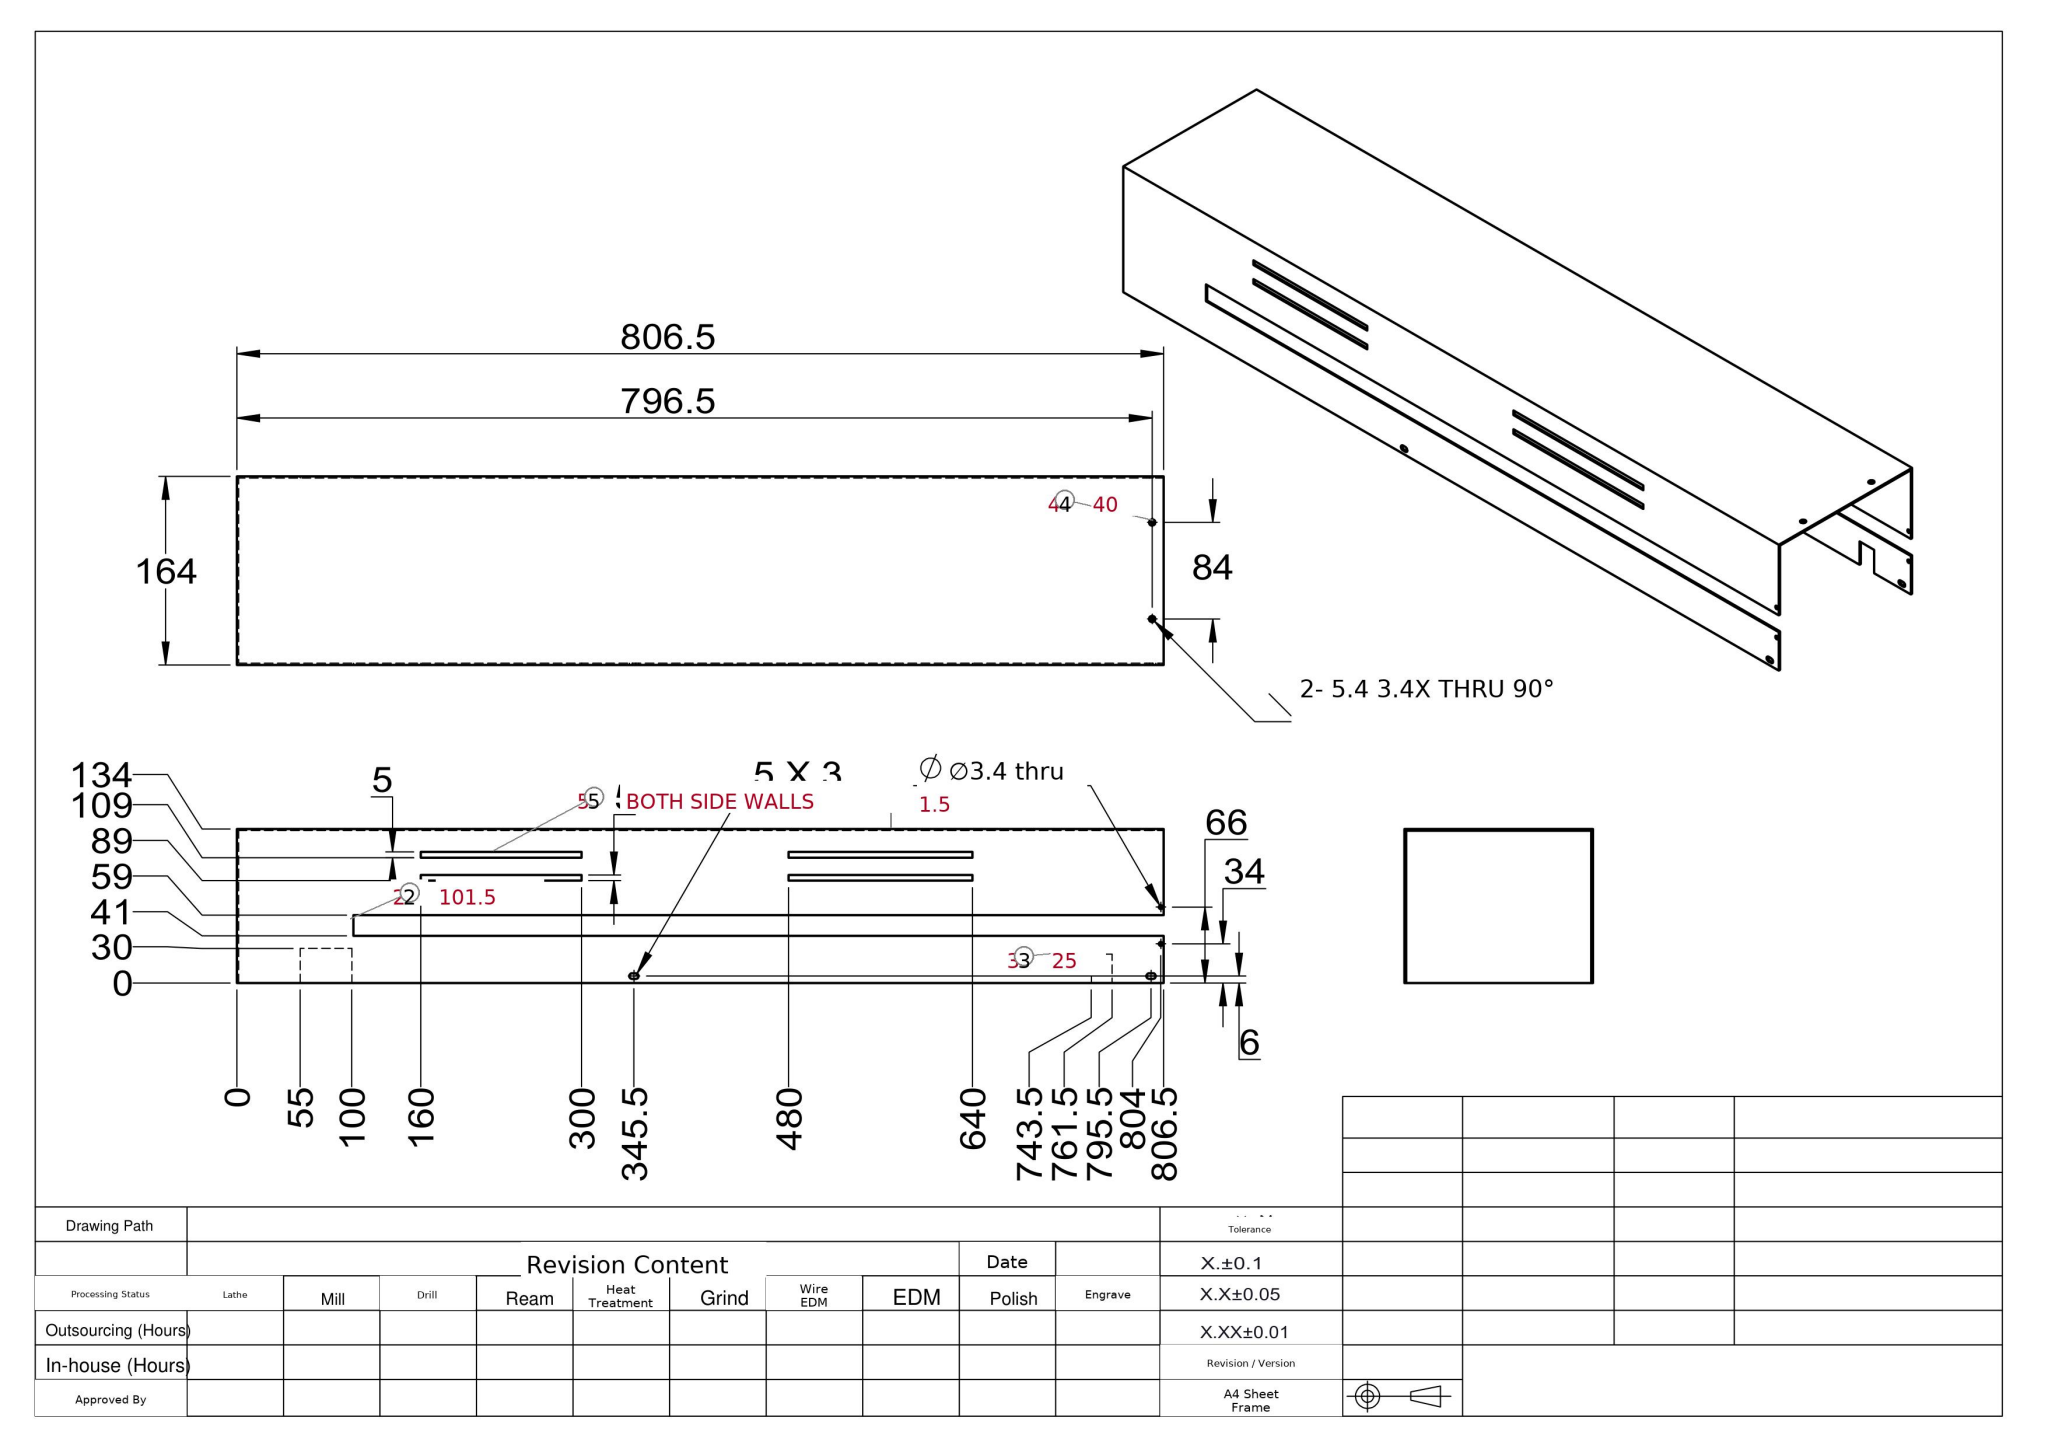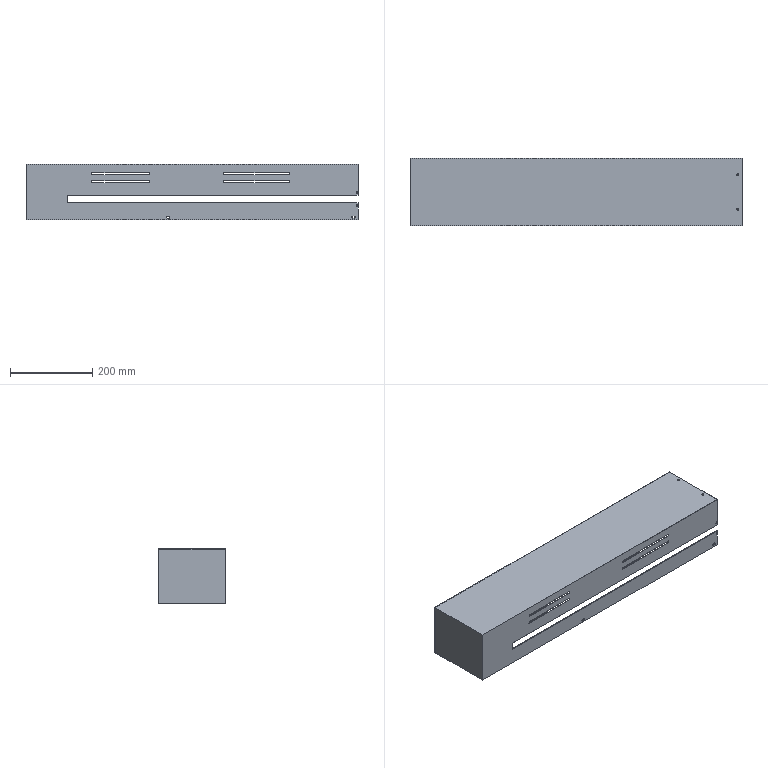Part | SolidWorks | mm | 1 solid | 90 faces | box 806.5 x 164 x 134 mm | volume 500909 mm3 | plane 66 | cylinder 20 | cone 4 | commonest cylinder face diameters 3.4 x12 5 x8
build123d program:
from build123d import *

# Parameters (mm, degrees)
SKETCH1_W           = 806.5
SKETCH1_H           = 164
BOSS_EXTRUDE1_DEPTH = 134
SKETCH2_W           = 805
SKETCH2_H           = 161
CUT_EXTRUDE1_DEPTH  = 834.843
SKETCH3_W           = 806.5
SKETCH3_H           = 164
BOSS_EXTRUDE2_DEPTH = 1.5
SKETCH4_W           = 705
SKETCH4_H           = 18
CUT_EXTRUDE2_DEPTH  = 834.843
SKETCH5_W           = 800
SKETCH5_H           = 5
CUT_EXTRUDE3_DEPTH  = 834.843
LPATTERN1_COUNT     = 2
LPATTERN1_PITCH     = 20
CUT_EXTRUDE4_DEPTH  = 834.843
LPATTERN2_COUNT     = 3
LPATTERN2_PITCH     = 450
SKETCH8_R           = 1.7
CUT_EXTRUDE5_DEPTH  = 1.5
CHAMFER1_SIZE       = 1
SKETCH9_W           = 45
SKETCH9_H           = 30
CUT_EXTRUDE6_DEPTH  = 10
SKETCH10_W          = 18
SKETCH10_H          = 25
CUT_EXTRUDE7_DEPTH  = 10
SKETCH11_W          = 180
SKETCH11_H          = 25
SKETCH11_W_2        = 166.5
BOSS_EXTRUDE4_DEPTH = 1.5
SKETCH12_W          = 180
SKETCH12_H          = 25
SKETCH12_W_2        = 166.5
BOSS_EXTRUDE5_DEPTH = 1.5
SKETCH14_R          = 1.7
CUT_EXTRUDE8_DEPTH  = 834.843


with BuildPart() as part:
    # Sketch1 → Boss-Extrude1 (new body)
    with BuildSketch(Plane.XY):
        with Locations((403.25, 82)):
            Rectangle(SKETCH1_W, SKETCH1_H)
    extrude(amount=BOSS_EXTRUDE1_DEPTH)

    # Sketch2 → Cut-Extrude1 (cut, through all)
    with BuildSketch(Plane.XY.offset(134)):
        with Locations((404, 82)):
            Rectangle(SKETCH2_W, SKETCH2_H)
    extrude(amount=-CUT_EXTRUDE1_DEPTH, mode=Mode.SUBTRACT)

    # Sketch3 → Boss-Extrude2 (add)
    with BuildSketch(Plane.XY.offset(134)):
        with Locations((403.25, 82)):
            Rectangle(SKETCH3_W, SKETCH3_H)
    extrude(amount=-BOSS_EXTRUDE2_DEPTH)

    # Sketch4 → Cut-Extrude2 (cut, through all)
    with BuildSketch(Plane(origin=(0, 164, 0), x_dir=(1, 0, 0), z_dir=(0, 1, 0))):
        with Locations((454, -50)):
            Rectangle(SKETCH4_W, SKETCH4_H)
    extrude(amount=-CUT_EXTRUDE2_DEPTH, mode=Mode.SUBTRACT)

    # Sketch5 → Cut-Extrude3 (cut, through all)
    with BuildSketch(Plane.XZ):
        with Locations((560, 111.5)):
            Rectangle(SKETCH5_W, SKETCH5_H)
    cut_extrude3 = extrude(amount=-CUT_EXTRUDE3_DEPTH, mode=Mode.SUBTRACT)

    # LPattern1: Cut-Extrude3 ×2
    with Locations(*[(0, 0, -i * LPATTERN1_PITCH) for i in range(1, LPATTERN1_COUNT)]):
        add(cut_extrude3, mode=Mode.SUBTRACT)

    # Sketch6 → Cut-Extrude4 (cut, through all)
    with BuildSketch(Plane.XZ):
        with BuildLine():
            Line((797, 3.5), (794, 3.5))
            ThreePointArc((794, 3.5), (791.5, 6), (794, 8.5))
            Line((794, 8.5), (797, 8.5))
            ThreePointArc((797, 8.5), (799.5, 6), (797, 3.5))
        make_face()
    cut_extrude4 = extrude(amount=-CUT_EXTRUDE4_DEPTH, mode=Mode.SUBTRACT)

    # LPattern2: Cut-Extrude4 ×3
    with Locations(*[(-i * LPATTERN2_PITCH, 0, 0) for i in range(1, LPATTERN2_COUNT)]):
        add(cut_extrude4, mode=Mode.SUBTRACT)

    # Sketch8 → Cut-Extrude5 (cut)
    with BuildSketch(Plane.XY.offset(134)):
        with Locations((796.5, 124)):
            Circle(SKETCH8_R)
        with Locations((796.5, 40)):
            Circle(SKETCH8_R)
    extrude(amount=-CUT_EXTRUDE5_DEPTH, mode=Mode.SUBTRACT)

    # Chamfer1
    chamfer1_edges = [part.edges().sort_by_distance(p)[0] for p in [
        (794.8, 124, 134),
        (794.8, 40, 134),
    ]]
    chamfer(chamfer1_edges, length=CHAMFER1_SIZE)

    # Sketch9 → Cut-Extrude6 (cut)
    with BuildSketch(Plane(origin=(0, 164, 0), x_dir=(1, 0, 0), z_dir=(0, 1, 0))):
        with Locations((77.5, -15)):
            Rectangle(SKETCH9_W, SKETCH9_H)
    extrude(amount=-CUT_EXTRUDE6_DEPTH, mode=Mode.SUBTRACT)

    # Sketch10 → Cut-Extrude7 (cut)
    with BuildSketch(Plane(origin=(0, 164, 0), x_dir=(1, 0, 0), z_dir=(0, 1, 0))):
        with Locations((752.5, -12.5)):
            Rectangle(SKETCH10_W, SKETCH10_H)
    extrude(amount=-CUT_EXTRUDE7_DEPTH, mode=Mode.SUBTRACT)

    # Sketch11 → Boss-Extrude4 (add)
    with BuildSketch(Plane(origin=(0, 164, 0), x_dir=(1, 0, 0), z_dir=(0, 1, 0))):
        with Locations((390, -101.5)):
            Rectangle(SKETCH11_W, SKETCH11_H)
        with Locations((723.25, -101.5)):
            Rectangle(SKETCH11_W_2, SKETCH11_H)
    extrude(amount=-BOSS_EXTRUDE4_DEPTH)

    # Sketch12 → Boss-Extrude5 (add)
    with BuildSketch(Plane.XZ):
        with Locations((390, 101.5)):
            Rectangle(SKETCH12_W, SKETCH12_H)
        with Locations((723.25, 101.5)):
            Rectangle(SKETCH12_W_2, SKETCH12_H)
    extrude(amount=-BOSS_EXTRUDE5_DEPTH)

    # Sketch14 → Cut-Extrude8 (cut, through all)
    with BuildSketch(Plane(origin=(0, 164, 0), x_dir=(1, 0, 0), z_dir=(0, 1, 0))):
        with Locations(Location((804, -66, 0), (0, 0, 270))):
            Circle(SKETCH14_R)
        with Locations(Location((804, -34, 0), (0, 0, 270))):
            Circle(SKETCH14_R)
    extrude(amount=-CUT_EXTRUDE8_DEPTH, mode=Mode.SUBTRACT)


solid = part.part